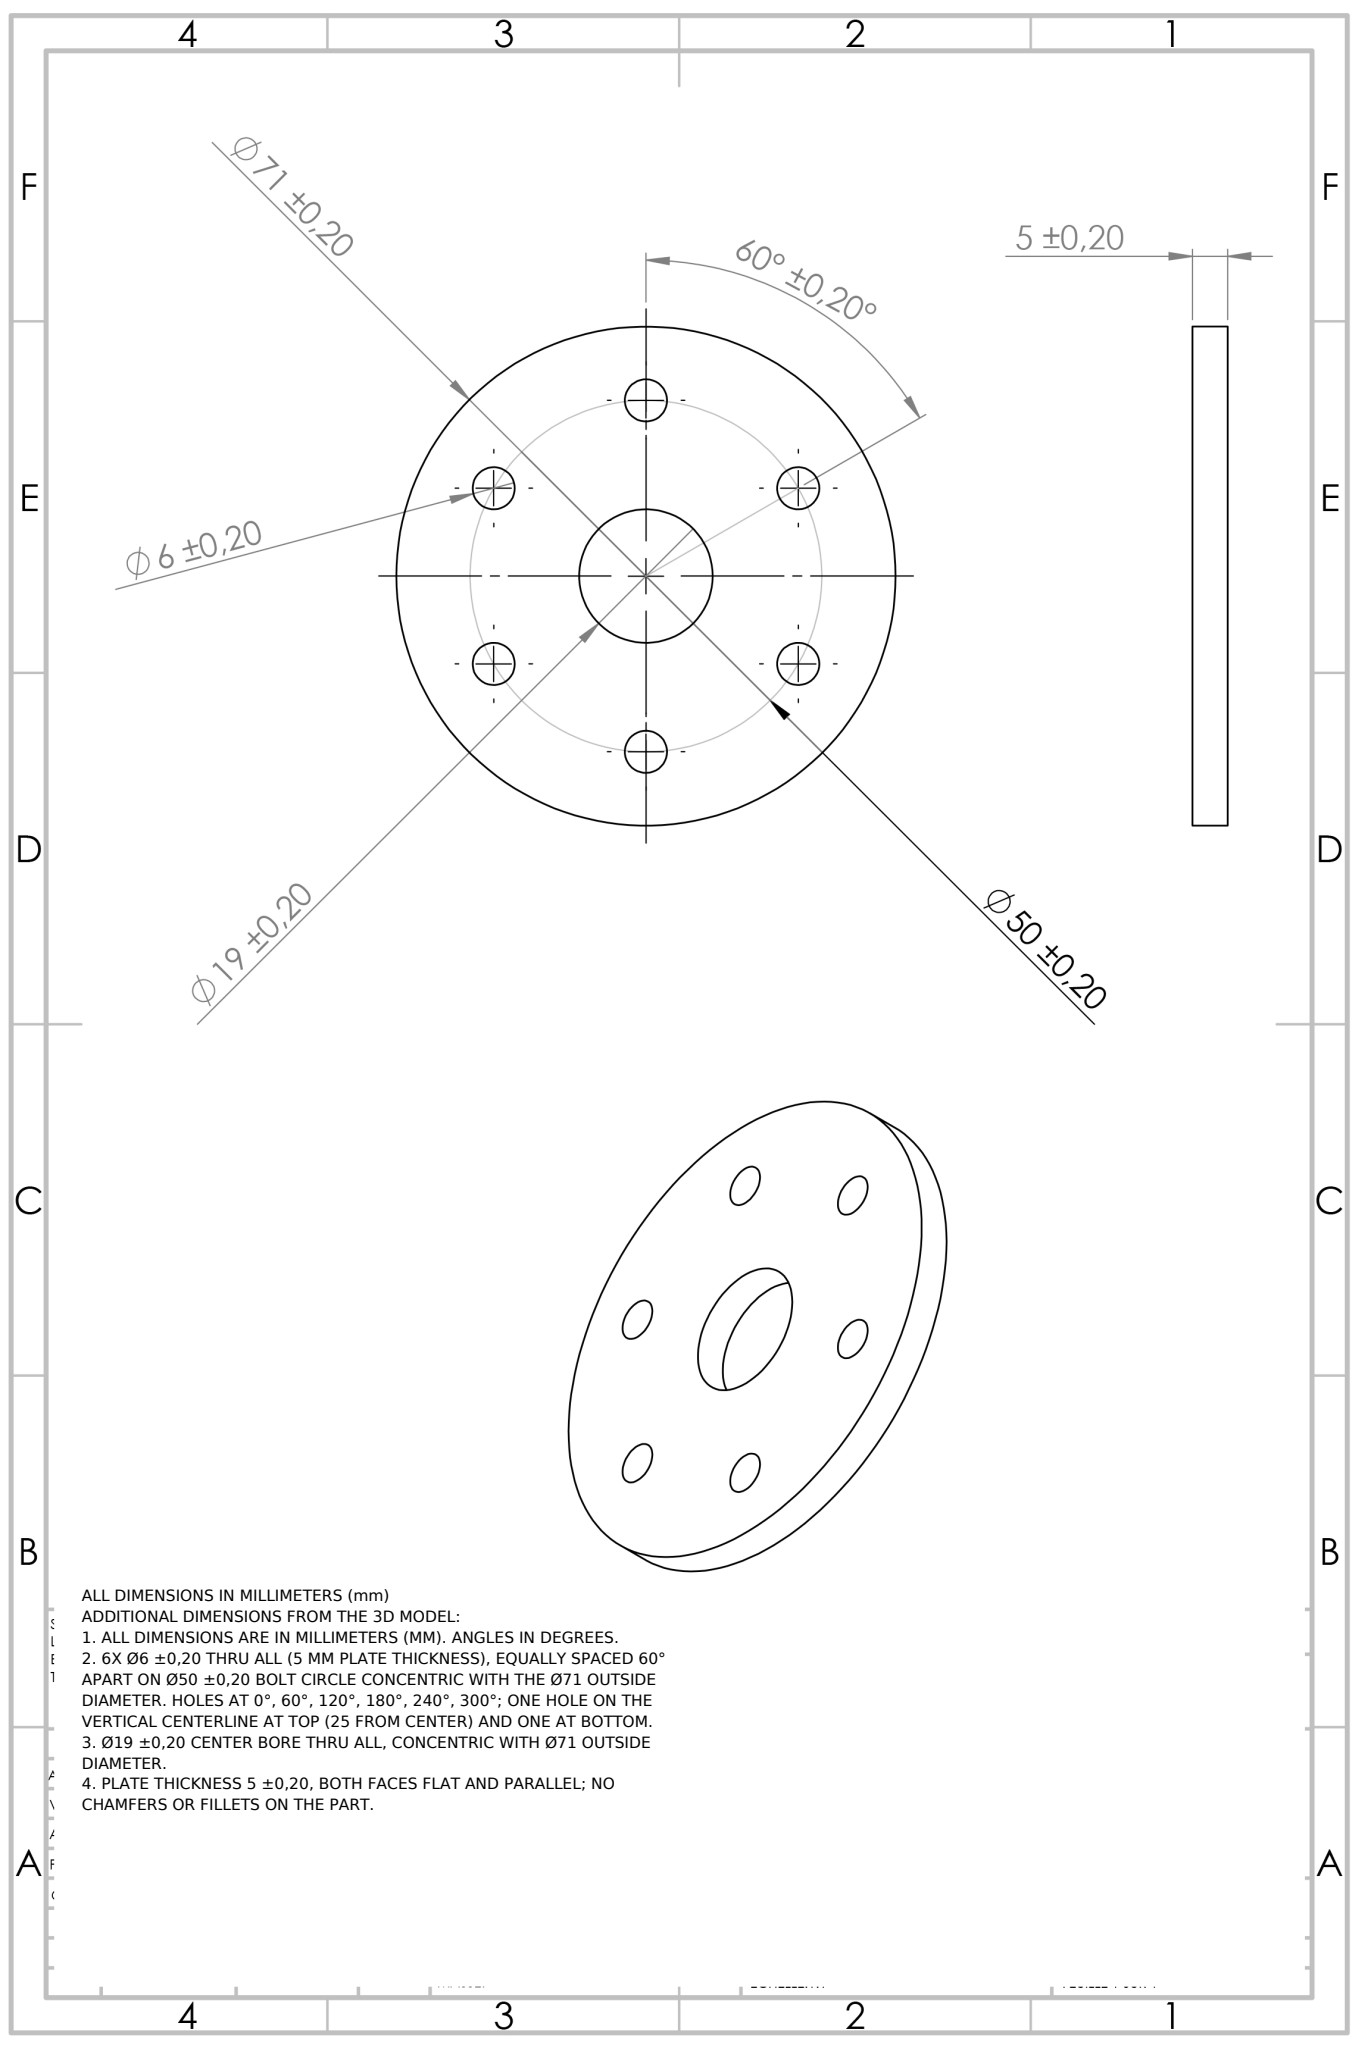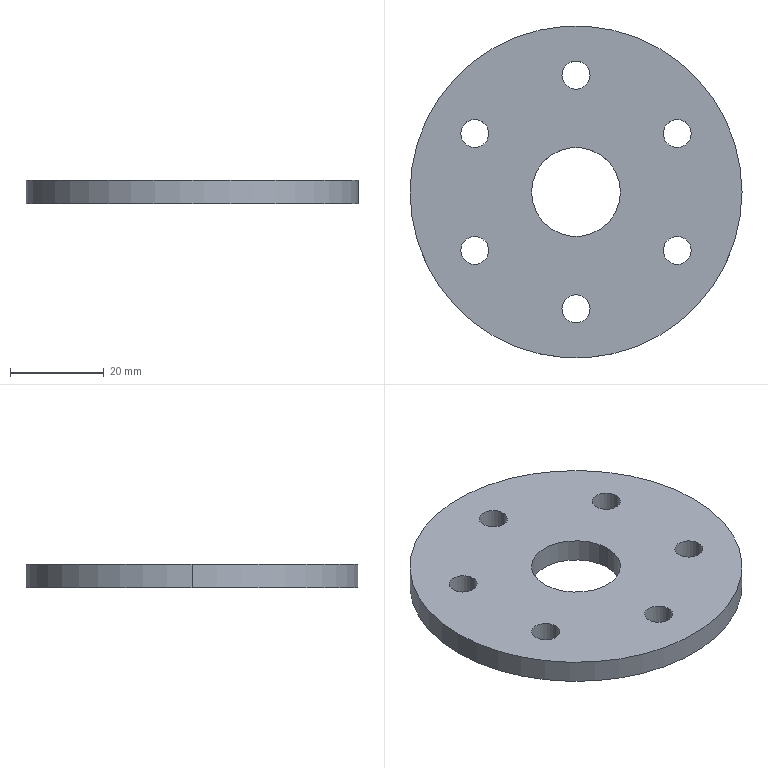Part | NX | mm | 1 solid | 18 faces | box 71 x 71 x 5 mm | volume 17530 mm3 | cylinder 16 | plane 2 | commonest cylinder face diameters 6 x12 19 x2 71 x2
STEP:
#1=COLOUR_RGB('',0.7922,0.8196,0.9333);
#2=FILL_AREA_STYLE_COLOUR('',#1);
#3=FILL_AREA_STYLE('',(#2));
#4=SURFACE_STYLE_FILL_AREA(#3);
#5=SURFACE_SIDE_STYLE('',(#4));
#6=SURFACE_STYLE_USAGE(.BOTH.,#5);
#7=PRESENTATION_STYLE_ASSIGNMENT((#6));
#8=CARTESIAN_POINT('',(-24.651,12.5,5.));
#9=VERTEX_POINT('',#8);
#10=CARTESIAN_POINT('',(-18.651,12.5,5.));
#11=VERTEX_POINT('',#10);
#12=CARTESIAN_POINT('',(-21.651,12.5,5.));
#13=DIRECTION('',(0.,0.,1.));
#14=DIRECTION('',(1.,0.,0.));
#15=AXIS2_PLACEMENT_3D('',#12,#13,#14);
#16=CIRCLE('',#15,3.);
#17=EDGE_CURVE('',#9,#11,#16,.T.);
#18=ORIENTED_EDGE('',*,*,#17,.T.);
#19=CARTESIAN_POINT('',(-18.651,12.5,0.));
#20=VERTEX_POINT('',#19);
#21=CARTESIAN_POINT('',(-18.651,12.5,5.));
#22=DIRECTION('',(0.,0.,-1.));
#23=VECTOR('',#22,1000.);
#24=LINE('',#21,#23);
#25=EDGE_CURVE('',#11,#20,#24,.T.);
#26=ORIENTED_EDGE('',*,*,#25,.T.);
#27=CARTESIAN_POINT('',(-24.651,12.5,0.));
#28=VERTEX_POINT('',#27);
#29=CARTESIAN_POINT('',(-21.651,12.5,0.));
#30=DIRECTION('',(0.,0.,1.));
#31=DIRECTION('',(1.,0.,0.));
#32=AXIS2_PLACEMENT_3D('',#29,#30,#31);
#33=CIRCLE('',#32,3.);
#34=EDGE_CURVE('',#28,#20,#33,.T.);
#35=ORIENTED_EDGE('',*,*,#34,.F.);
#36=CARTESIAN_POINT('',(-24.651,12.5,5.));
#37=DIRECTION('',(0.,0.,-1.));
#38=VECTOR('',#37,1000.);
#39=LINE('',#36,#38);
#40=EDGE_CURVE('',#9,#28,#39,.T.);
#41=ORIENTED_EDGE('',*,*,#40,.F.);
#42=EDGE_LOOP('',(#18,#26,#35,#41));
#43=FACE_OUTER_BOUND('',#42,.T.);
#44=CARTESIAN_POINT('',(-21.651,12.5,5.));
#45=DIRECTION('',(0.,0.,-1.));
#46=DIRECTION('',(-1.,0.,0.));
#47=AXIS2_PLACEMENT_3D('',#44,#45,#46);
#48=CYLINDRICAL_SURFACE('',#47,3.);
#49=ADVANCED_FACE('',(#43),#48,.F.);
#50=CARTESIAN_POINT('',(-24.651,-12.5,5.));
#51=VERTEX_POINT('',#50);
#52=CARTESIAN_POINT('',(-18.651,-12.5,5.));
#53=VERTEX_POINT('',#52);
#54=CARTESIAN_POINT('',(-21.651,-12.5,5.));
#55=DIRECTION('',(0.,0.,1.));
#56=DIRECTION('',(1.,0.,0.));
#57=AXIS2_PLACEMENT_3D('',#54,#55,#56);
#58=CIRCLE('',#57,3.);
#59=EDGE_CURVE('',#51,#53,#58,.T.);
#60=ORIENTED_EDGE('',*,*,#59,.T.);
#61=CARTESIAN_POINT('',(-18.651,-12.5,0.));
#62=VERTEX_POINT('',#61);
#63=CARTESIAN_POINT('',(-18.651,-12.5,5.));
#64=DIRECTION('',(0.,0.,-1.));
#65=VECTOR('',#64,1000.);
#66=LINE('',#63,#65);
#67=EDGE_CURVE('',#53,#62,#66,.T.);
#68=ORIENTED_EDGE('',*,*,#67,.T.);
#69=CARTESIAN_POINT('',(-24.651,-12.5,0.));
#70=VERTEX_POINT('',#69);
#71=CARTESIAN_POINT('',(-21.651,-12.5,0.));
#72=DIRECTION('',(0.,0.,1.));
#73=DIRECTION('',(1.,0.,0.));
#74=AXIS2_PLACEMENT_3D('',#71,#72,#73);
#75=CIRCLE('',#74,3.);
#76=EDGE_CURVE('',#70,#62,#75,.T.);
#77=ORIENTED_EDGE('',*,*,#76,.F.);
#78=CARTESIAN_POINT('',(-24.651,-12.5,5.));
#79=DIRECTION('',(0.,0.,-1.));
#80=VECTOR('',#79,1000.);
#81=LINE('',#78,#80);
#82=EDGE_CURVE('',#51,#70,#81,.T.);
#83=ORIENTED_EDGE('',*,*,#82,.F.);
#84=EDGE_LOOP('',(#60,#68,#77,#83));
#85=FACE_OUTER_BOUND('',#84,.T.);
#86=CARTESIAN_POINT('',(-21.651,-12.5,5.));
#87=DIRECTION('',(0.,0.,-1.));
#88=DIRECTION('',(-1.,0.,0.));
#89=AXIS2_PLACEMENT_3D('',#86,#87,#88);
#90=CYLINDRICAL_SURFACE('',#89,3.);
#91=ADVANCED_FACE('',(#85),#90,.F.);
#92=CARTESIAN_POINT('',(-3.,-25.,5.));
#93=VERTEX_POINT('',#92);
#94=CARTESIAN_POINT('',(3.,-25.,5.));
#95=VERTEX_POINT('',#94);
#96=CARTESIAN_POINT('',(0.,-25.,5.));
#97=DIRECTION('',(0.,0.,1.));
#98=DIRECTION('',(1.,0.,0.));
#99=AXIS2_PLACEMENT_3D('',#96,#97,#98);
#100=CIRCLE('',#99,3.);
#101=EDGE_CURVE('',#93,#95,#100,.T.);
#102=ORIENTED_EDGE('',*,*,#101,.T.);
#103=CARTESIAN_POINT('',(3.,-25.,0.));
#104=VERTEX_POINT('',#103);
#105=CARTESIAN_POINT('',(3.,-25.,5.));
#106=DIRECTION('',(0.,0.,-1.));
#107=VECTOR('',#106,1000.);
#108=LINE('',#105,#107);
#109=EDGE_CURVE('',#95,#104,#108,.T.);
#110=ORIENTED_EDGE('',*,*,#109,.T.);
#111=CARTESIAN_POINT('',(-3.,-25.,0.));
#112=VERTEX_POINT('',#111);
#113=CARTESIAN_POINT('',(0.,-25.,0.));
#114=DIRECTION('',(0.,0.,1.));
#115=DIRECTION('',(1.,0.,0.));
#116=AXIS2_PLACEMENT_3D('',#113,#114,#115);
#117=CIRCLE('',#116,3.);
#118=EDGE_CURVE('',#112,#104,#117,.T.);
#119=ORIENTED_EDGE('',*,*,#118,.F.);
#120=CARTESIAN_POINT('',(-3.,-25.,5.));
#121=DIRECTION('',(0.,0.,-1.));
#122=VECTOR('',#121,1000.);
#123=LINE('',#120,#122);
#124=EDGE_CURVE('',#93,#112,#123,.T.);
#125=ORIENTED_EDGE('',*,*,#124,.F.);
#126=EDGE_LOOP('',(#102,#110,#119,#125));
#127=FACE_OUTER_BOUND('',#126,.T.);
#128=CARTESIAN_POINT('',(0.,-25.,5.));
#129=DIRECTION('',(0.,0.,-1.));
#130=DIRECTION('',(-1.,0.,0.));
#131=AXIS2_PLACEMENT_3D('',#128,#129,#130);
#132=CYLINDRICAL_SURFACE('',#131,3.);
#133=ADVANCED_FACE('',(#127),#132,.F.);
#134=CARTESIAN_POINT('',(18.651,-12.5,5.));
#135=VERTEX_POINT('',#134);
#136=CARTESIAN_POINT('',(24.651,-12.5,5.));
#137=VERTEX_POINT('',#136);
#138=CARTESIAN_POINT('',(21.651,-12.5,5.));
#139=DIRECTION('',(0.,0.,1.));
#140=DIRECTION('',(1.,0.,0.));
#141=AXIS2_PLACEMENT_3D('',#138,#139,#140);
#142=CIRCLE('',#141,3.);
#143=EDGE_CURVE('',#135,#137,#142,.T.);
#144=ORIENTED_EDGE('',*,*,#143,.T.);
#145=CARTESIAN_POINT('',(24.651,-12.5,0.));
#146=VERTEX_POINT('',#145);
#147=CARTESIAN_POINT('',(24.651,-12.5,5.));
#148=DIRECTION('',(0.,0.,-1.));
#149=VECTOR('',#148,1000.);
#150=LINE('',#147,#149);
#151=EDGE_CURVE('',#137,#146,#150,.T.);
#152=ORIENTED_EDGE('',*,*,#151,.T.);
#153=CARTESIAN_POINT('',(18.651,-12.5,0.));
#154=VERTEX_POINT('',#153);
#155=CARTESIAN_POINT('',(21.651,-12.5,0.));
#156=DIRECTION('',(0.,0.,1.));
#157=DIRECTION('',(1.,0.,0.));
#158=AXIS2_PLACEMENT_3D('',#155,#156,#157);
#159=CIRCLE('',#158,3.);
#160=EDGE_CURVE('',#154,#146,#159,.T.);
#161=ORIENTED_EDGE('',*,*,#160,.F.);
#162=CARTESIAN_POINT('',(18.651,-12.5,5.));
#163=DIRECTION('',(0.,0.,-1.));
#164=VECTOR('',#163,1000.);
#165=LINE('',#162,#164);
#166=EDGE_CURVE('',#135,#154,#165,.T.);
#167=ORIENTED_EDGE('',*,*,#166,.F.);
#168=EDGE_LOOP('',(#144,#152,#161,#167));
#169=FACE_OUTER_BOUND('',#168,.T.);
#170=CARTESIAN_POINT('',(21.651,-12.5,5.));
#171=DIRECTION('',(0.,0.,-1.));
#172=DIRECTION('',(-1.,0.,0.));
#173=AXIS2_PLACEMENT_3D('',#170,#171,#172);
#174=CYLINDRICAL_SURFACE('',#173,3.);
#175=ADVANCED_FACE('',(#169),#174,.F.);
#176=CARTESIAN_POINT('',(18.651,12.5,5.));
#177=VERTEX_POINT('',#176);
#178=CARTESIAN_POINT('',(24.651,12.5,5.));
#179=VERTEX_POINT('',#178);
#180=CARTESIAN_POINT('',(21.651,12.5,5.));
#181=DIRECTION('',(0.,0.,1.));
#182=DIRECTION('',(1.,0.,0.));
#183=AXIS2_PLACEMENT_3D('',#180,#181,#182);
#184=CIRCLE('',#183,3.);
#185=EDGE_CURVE('',#177,#179,#184,.T.);
#186=ORIENTED_EDGE('',*,*,#185,.T.);
#187=CARTESIAN_POINT('',(24.651,12.5,0.));
#188=VERTEX_POINT('',#187);
#189=CARTESIAN_POINT('',(24.651,12.5,5.));
#190=DIRECTION('',(0.,0.,-1.));
#191=VECTOR('',#190,1000.);
#192=LINE('',#189,#191);
#193=EDGE_CURVE('',#179,#188,#192,.T.);
#194=ORIENTED_EDGE('',*,*,#193,.T.);
#195=CARTESIAN_POINT('',(18.651,12.5,0.));
#196=VERTEX_POINT('',#195);
#197=CARTESIAN_POINT('',(21.651,12.5,0.));
#198=DIRECTION('',(0.,0.,1.));
#199=DIRECTION('',(1.,0.,0.));
#200=AXIS2_PLACEMENT_3D('',#197,#198,#199);
#201=CIRCLE('',#200,3.);
#202=EDGE_CURVE('',#196,#188,#201,.T.);
#203=ORIENTED_EDGE('',*,*,#202,.F.);
#204=CARTESIAN_POINT('',(18.651,12.5,5.));
#205=DIRECTION('',(0.,0.,-1.));
#206=VECTOR('',#205,1000.);
#207=LINE('',#204,#206);
#208=EDGE_CURVE('',#177,#196,#207,.T.);
#209=ORIENTED_EDGE('',*,*,#208,.F.);
#210=EDGE_LOOP('',(#186,#194,#203,#209));
#211=FACE_OUTER_BOUND('',#210,.T.);
#212=CARTESIAN_POINT('',(21.651,12.5,5.));
#213=DIRECTION('',(0.,0.,-1.));
#214=DIRECTION('',(-1.,0.,0.));
#215=AXIS2_PLACEMENT_3D('',#212,#213,#214);
#216=CYLINDRICAL_SURFACE('',#215,3.);
#217=ADVANCED_FACE('',(#211),#216,.F.);
#218=CARTESIAN_POINT('',(-3.,25.,5.));
#219=VERTEX_POINT('',#218);
#220=CARTESIAN_POINT('',(3.,25.,5.));
#221=VERTEX_POINT('',#220);
#222=CARTESIAN_POINT('',(0.,25.,5.));
#223=DIRECTION('',(0.,0.,1.));
#224=DIRECTION('',(1.,0.,0.));
#225=AXIS2_PLACEMENT_3D('',#222,#223,#224);
#226=CIRCLE('',#225,3.);
#227=EDGE_CURVE('',#219,#221,#226,.T.);
#228=ORIENTED_EDGE('',*,*,#227,.T.);
#229=CARTESIAN_POINT('',(3.,25.,0.));
#230=VERTEX_POINT('',#229);
#231=CARTESIAN_POINT('',(3.,25.,5.));
#232=DIRECTION('',(0.,0.,-1.));
#233=VECTOR('',#232,1000.);
#234=LINE('',#231,#233);
#235=EDGE_CURVE('',#221,#230,#234,.T.);
#236=ORIENTED_EDGE('',*,*,#235,.T.);
#237=CARTESIAN_POINT('',(-3.,25.,0.));
#238=VERTEX_POINT('',#237);
#239=CARTESIAN_POINT('',(0.,25.,0.));
#240=DIRECTION('',(0.,0.,1.));
#241=DIRECTION('',(1.,0.,0.));
#242=AXIS2_PLACEMENT_3D('',#239,#240,#241);
#243=CIRCLE('',#242,3.);
#244=EDGE_CURVE('',#238,#230,#243,.T.);
#245=ORIENTED_EDGE('',*,*,#244,.F.);
#246=CARTESIAN_POINT('',(-3.,25.,5.));
#247=DIRECTION('',(0.,0.,-1.));
#248=VECTOR('',#247,1000.);
#249=LINE('',#246,#248);
#250=EDGE_CURVE('',#219,#238,#249,.T.);
#251=ORIENTED_EDGE('',*,*,#250,.F.);
#252=EDGE_LOOP('',(#228,#236,#245,#251));
#253=FACE_OUTER_BOUND('',#252,.T.);
#254=CARTESIAN_POINT('',(0.,25.,5.));
#255=DIRECTION('',(0.,0.,-1.));
#256=DIRECTION('',(-1.,0.,0.));
#257=AXIS2_PLACEMENT_3D('',#254,#255,#256);
#258=CYLINDRICAL_SURFACE('',#257,3.);
#259=ADVANCED_FACE('',(#253),#258,.F.);
#260=CARTESIAN_POINT('',(-9.5,0.,5.));
#261=VERTEX_POINT('',#260);
#262=CARTESIAN_POINT('',(9.5,0.,5.));
#263=VERTEX_POINT('',#262);
#264=CARTESIAN_POINT('',(0.,0.,5.));
#265=DIRECTION('',(0.,0.,1.));
#266=DIRECTION('',(1.,0.,0.));
#267=AXIS2_PLACEMENT_3D('',#264,#265,#266);
#268=CIRCLE('',#267,9.5);
#269=EDGE_CURVE('',#261,#263,#268,.T.);
#270=ORIENTED_EDGE('',*,*,#269,.T.);
#271=CARTESIAN_POINT('',(9.5,0.,0.));
#272=VERTEX_POINT('',#271);
#273=CARTESIAN_POINT('',(9.5,0.,5.));
#274=DIRECTION('',(0.,0.,-1.));
#275=VECTOR('',#274,1000.);
#276=LINE('',#273,#275);
#277=EDGE_CURVE('',#263,#272,#276,.T.);
#278=ORIENTED_EDGE('',*,*,#277,.T.);
#279=CARTESIAN_POINT('',(-9.5,0.,0.));
#280=VERTEX_POINT('',#279);
#281=CARTESIAN_POINT('',(0.,0.,0.));
#282=DIRECTION('',(0.,0.,1.));
#283=DIRECTION('',(1.,0.,0.));
#284=AXIS2_PLACEMENT_3D('',#281,#282,#283);
#285=CIRCLE('',#284,9.5);
#286=EDGE_CURVE('',#280,#272,#285,.T.);
#287=ORIENTED_EDGE('',*,*,#286,.F.);
#288=CARTESIAN_POINT('',(-9.5,0.,5.));
#289=DIRECTION('',(0.,0.,-1.));
#290=VECTOR('',#289,1000.);
#291=LINE('',#288,#290);
#292=EDGE_CURVE('',#261,#280,#291,.T.);
#293=ORIENTED_EDGE('',*,*,#292,.F.);
#294=EDGE_LOOP('',(#270,#278,#287,#293));
#295=FACE_OUTER_BOUND('',#294,.T.);
#296=CARTESIAN_POINT('',(0.,0.,5.));
#297=DIRECTION('',(0.,0.,-1.));
#298=DIRECTION('',(-1.,0.,0.));
#299=AXIS2_PLACEMENT_3D('',#296,#297,#298);
#300=CYLINDRICAL_SURFACE('',#299,9.5);
#301=ADVANCED_FACE('',(#295),#300,.F.);
#302=CARTESIAN_POINT('',(35.5,0.,5.));
#303=VERTEX_POINT('',#302);
#304=CARTESIAN_POINT('',(-35.5,0.,5.));
#305=VERTEX_POINT('',#304);
#306=CARTESIAN_POINT('',(0.,0.,5.));
#307=DIRECTION('',(0.,0.,1.));
#308=DIRECTION('',(1.,0.,0.));
#309=AXIS2_PLACEMENT_3D('',#306,#307,#308);
#310=CIRCLE('',#309,35.5);
#311=EDGE_CURVE('',#303,#305,#310,.T.);
#312=ORIENTED_EDGE('',*,*,#311,.F.);
#313=CARTESIAN_POINT('',(35.5,0.,0.));
#314=VERTEX_POINT('',#313);
#315=CARTESIAN_POINT('',(35.5,0.,5.));
#316=DIRECTION('',(0.,0.,-1.));
#317=VECTOR('',#316,1000.);
#318=LINE('',#315,#317);
#319=EDGE_CURVE('',#303,#314,#318,.T.);
#320=ORIENTED_EDGE('',*,*,#319,.T.);
#321=CARTESIAN_POINT('',(-35.5,0.,0.));
#322=VERTEX_POINT('',#321);
#323=CARTESIAN_POINT('',(0.,0.,0.));
#324=DIRECTION('',(0.,0.,1.));
#325=DIRECTION('',(1.,0.,0.));
#326=AXIS2_PLACEMENT_3D('',#323,#324,#325);
#327=CIRCLE('',#326,35.5);
#328=EDGE_CURVE('',#314,#322,#327,.T.);
#329=ORIENTED_EDGE('',*,*,#328,.T.);
#330=CARTESIAN_POINT('',(-35.5,0.,5.));
#331=DIRECTION('',(0.,0.,-1.));
#332=VECTOR('',#331,1000.);
#333=LINE('',#330,#332);
#334=EDGE_CURVE('',#305,#322,#333,.T.);
#335=ORIENTED_EDGE('',*,*,#334,.F.);
#336=EDGE_LOOP('',(#312,#320,#329,#335));
#337=FACE_OUTER_BOUND('',#336,.T.);
#338=CARTESIAN_POINT('',(0.,0.,5.));
#339=DIRECTION('',(0.,0.,-1.));
#340=DIRECTION('',(-1.,0.,0.));
#341=AXIS2_PLACEMENT_3D('',#338,#339,#340);
#342=CYLINDRICAL_SURFACE('',#341,35.5);
#343=ADVANCED_FACE('',(#337),#342,.T.);
#344=ORIENTED_EDGE('',*,*,#59,.F.);
#345=CARTESIAN_POINT('',(-21.651,-12.5,5.));
#346=DIRECTION('',(0.,0.,1.));
#347=DIRECTION('',(1.,0.,0.));
#348=AXIS2_PLACEMENT_3D('',#345,#346,#347);
#349=CIRCLE('',#348,3.);
#350=EDGE_CURVE('',#53,#51,#349,.T.);
#351=ORIENTED_EDGE('',*,*,#350,.F.);
#352=EDGE_LOOP('',(#344,#351));
#353=FACE_BOUND('',#352,.T.);
#354=ORIENTED_EDGE('',*,*,#143,.F.);
#355=CARTESIAN_POINT('',(21.651,-12.5,5.));
#356=DIRECTION('',(0.,0.,1.));
#357=DIRECTION('',(1.,0.,0.));
#358=AXIS2_PLACEMENT_3D('',#355,#356,#357);
#359=CIRCLE('',#358,3.);
#360=EDGE_CURVE('',#137,#135,#359,.T.);
#361=ORIENTED_EDGE('',*,*,#360,.F.);
#362=EDGE_LOOP('',(#354,#361));
#363=FACE_BOUND('',#362,.T.);
#364=ORIENTED_EDGE('',*,*,#227,.F.);
#365=CARTESIAN_POINT('',(0.,25.,5.));
#366=DIRECTION('',(0.,0.,1.));
#367=DIRECTION('',(1.,0.,0.));
#368=AXIS2_PLACEMENT_3D('',#365,#366,#367);
#369=CIRCLE('',#368,3.);
#370=EDGE_CURVE('',#221,#219,#369,.T.);
#371=ORIENTED_EDGE('',*,*,#370,.F.);
#372=EDGE_LOOP('',(#364,#371));
#373=FACE_BOUND('',#372,.T.);
#374=CARTESIAN_POINT('',(0.,0.,5.));
#375=DIRECTION('',(0.,0.,1.));
#376=DIRECTION('',(1.,0.,0.));
#377=AXIS2_PLACEMENT_3D('',#374,#375,#376);
#378=CIRCLE('',#377,35.5);
#379=EDGE_CURVE('',#305,#303,#378,.T.);
#380=ORIENTED_EDGE('',*,*,#379,.T.);
#381=ORIENTED_EDGE('',*,*,#311,.T.);
#382=EDGE_LOOP('',(#380,#381));
#383=FACE_OUTER_BOUND('',#382,.T.);
#384=ORIENTED_EDGE('',*,*,#269,.F.);
#385=CARTESIAN_POINT('',(0.,0.,5.));
#386=DIRECTION('',(0.,0.,1.));
#387=DIRECTION('',(1.,0.,0.));
#388=AXIS2_PLACEMENT_3D('',#385,#386,#387);
#389=CIRCLE('',#388,9.5);
#390=EDGE_CURVE('',#263,#261,#389,.T.);
#391=ORIENTED_EDGE('',*,*,#390,.F.);
#392=EDGE_LOOP('',(#384,#391));
#393=FACE_BOUND('',#392,.T.);
#394=ORIENTED_EDGE('',*,*,#185,.F.);
#395=CARTESIAN_POINT('',(21.651,12.5,5.));
#396=DIRECTION('',(0.,0.,1.));
#397=DIRECTION('',(1.,0.,0.));
#398=AXIS2_PLACEMENT_3D('',#395,#396,#397);
#399=CIRCLE('',#398,3.);
#400=EDGE_CURVE('',#179,#177,#399,.T.);
#401=ORIENTED_EDGE('',*,*,#400,.F.);
#402=EDGE_LOOP('',(#394,#401));
#403=FACE_BOUND('',#402,.T.);
#404=ORIENTED_EDGE('',*,*,#101,.F.);
#405=CARTESIAN_POINT('',(0.,-25.,5.));
#406=DIRECTION('',(0.,0.,1.));
#407=DIRECTION('',(1.,0.,0.));
#408=AXIS2_PLACEMENT_3D('',#405,#406,#407);
#409=CIRCLE('',#408,3.);
#410=EDGE_CURVE('',#95,#93,#409,.T.);
#411=ORIENTED_EDGE('',*,*,#410,.F.);
#412=EDGE_LOOP('',(#404,#411));
#413=FACE_BOUND('',#412,.T.);
#414=ORIENTED_EDGE('',*,*,#17,.F.);
#415=CARTESIAN_POINT('',(-21.651,12.5,5.));
#416=DIRECTION('',(0.,0.,1.));
#417=DIRECTION('',(1.,0.,0.));
#418=AXIS2_PLACEMENT_3D('',#415,#416,#417);
#419=CIRCLE('',#418,3.);
#420=EDGE_CURVE('',#11,#9,#419,.T.);
#421=ORIENTED_EDGE('',*,*,#420,.F.);
#422=EDGE_LOOP('',(#414,#421));
#423=FACE_BOUND('',#422,.T.);
#424=CARTESIAN_POINT('',(0.,0.,5.));
#425=DIRECTION('',(0.,0.,1.));
#426=DIRECTION('',(1.,0.,0.));
#427=AXIS2_PLACEMENT_3D('',#424,#425,#426);
#428=PLANE('',#427);
#429=ADVANCED_FACE('',(#353,#363,#373,#383,#393,#403,#413,#423),#428,.T.);
#430=CARTESIAN_POINT('',(0.,0.,0.));
#431=DIRECTION('',(0.,0.,1.));
#432=DIRECTION('',(1.,0.,0.));
#433=AXIS2_PLACEMENT_3D('',#430,#431,#432);
#434=CIRCLE('',#433,35.5);
#435=EDGE_CURVE('',#322,#314,#434,.T.);
#436=ORIENTED_EDGE('',*,*,#435,.F.);
#437=ORIENTED_EDGE('',*,*,#328,.F.);
#438=EDGE_LOOP('',(#436,#437));
#439=FACE_OUTER_BOUND('',#438,.T.);
#440=ORIENTED_EDGE('',*,*,#286,.T.);
#441=CARTESIAN_POINT('',(0.,0.,0.));
#442=DIRECTION('',(0.,0.,1.));
#443=DIRECTION('',(1.,0.,0.));
#444=AXIS2_PLACEMENT_3D('',#441,#442,#443);
#445=CIRCLE('',#444,9.5);
#446=EDGE_CURVE('',#272,#280,#445,.T.);
#447=ORIENTED_EDGE('',*,*,#446,.T.);
#448=EDGE_LOOP('',(#440,#447));
#449=FACE_BOUND('',#448,.T.);
#450=ORIENTED_EDGE('',*,*,#244,.T.);
#451=CARTESIAN_POINT('',(0.,25.,0.));
#452=DIRECTION('',(0.,0.,1.));
#453=DIRECTION('',(1.,0.,0.));
#454=AXIS2_PLACEMENT_3D('',#451,#452,#453);
#455=CIRCLE('',#454,3.);
#456=EDGE_CURVE('',#230,#238,#455,.T.);
#457=ORIENTED_EDGE('',*,*,#456,.T.);
#458=EDGE_LOOP('',(#450,#457));
#459=FACE_BOUND('',#458,.T.);
#460=ORIENTED_EDGE('',*,*,#202,.T.);
#461=CARTESIAN_POINT('',(21.651,12.5,0.));
#462=DIRECTION('',(0.,0.,1.));
#463=DIRECTION('',(1.,0.,0.));
#464=AXIS2_PLACEMENT_3D('',#461,#462,#463);
#465=CIRCLE('',#464,3.);
#466=EDGE_CURVE('',#188,#196,#465,.T.);
#467=ORIENTED_EDGE('',*,*,#466,.T.);
#468=EDGE_LOOP('',(#460,#467));
#469=FACE_BOUND('',#468,.T.);
#470=ORIENTED_EDGE('',*,*,#160,.T.);
#471=CARTESIAN_POINT('',(21.651,-12.5,0.));
#472=DIRECTION('',(0.,0.,1.));
#473=DIRECTION('',(1.,0.,0.));
#474=AXIS2_PLACEMENT_3D('',#471,#472,#473);
#475=CIRCLE('',#474,3.);
#476=EDGE_CURVE('',#146,#154,#475,.T.);
#477=ORIENTED_EDGE('',*,*,#476,.T.);
#478=EDGE_LOOP('',(#470,#477));
#479=FACE_BOUND('',#478,.T.);
#480=ORIENTED_EDGE('',*,*,#118,.T.);
#481=CARTESIAN_POINT('',(0.,-25.,0.));
#482=DIRECTION('',(0.,0.,1.));
#483=DIRECTION('',(1.,0.,0.));
#484=AXIS2_PLACEMENT_3D('',#481,#482,#483);
#485=CIRCLE('',#484,3.);
#486=EDGE_CURVE('',#104,#112,#485,.T.);
#487=ORIENTED_EDGE('',*,*,#486,.T.);
#488=EDGE_LOOP('',(#480,#487));
#489=FACE_BOUND('',#488,.T.);
#490=ORIENTED_EDGE('',*,*,#76,.T.);
#491=CARTESIAN_POINT('',(-21.651,-12.5,0.));
#492=DIRECTION('',(0.,0.,1.));
#493=DIRECTION('',(1.,0.,0.));
#494=AXIS2_PLACEMENT_3D('',#491,#492,#493);
#495=CIRCLE('',#494,3.);
#496=EDGE_CURVE('',#62,#70,#495,.T.);
#497=ORIENTED_EDGE('',*,*,#496,.T.);
#498=EDGE_LOOP('',(#490,#497));
#499=FACE_BOUND('',#498,.T.);
#500=ORIENTED_EDGE('',*,*,#34,.T.);
#501=CARTESIAN_POINT('',(-21.651,12.5,0.));
#502=DIRECTION('',(0.,0.,1.));
#503=DIRECTION('',(1.,0.,0.));
#504=AXIS2_PLACEMENT_3D('',#501,#502,#503);
#505=CIRCLE('',#504,3.);
#506=EDGE_CURVE('',#20,#28,#505,.T.);
#507=ORIENTED_EDGE('',*,*,#506,.T.);
#508=EDGE_LOOP('',(#500,#507));
#509=FACE_BOUND('',#508,.T.);
#510=CARTESIAN_POINT('',(0.,0.,0.));
#511=DIRECTION('',(0.,0.,1.));
#512=DIRECTION('',(1.,0.,0.));
#513=AXIS2_PLACEMENT_3D('',#510,#511,#512);
#514=PLANE('',#513);
#515=ADVANCED_FACE('',(#439,#449,#459,#469,#479,#489,#499,#509),#514,.F.);
#516=ORIENTED_EDGE('',*,*,#319,.F.);
#517=ORIENTED_EDGE('',*,*,#379,.F.);
#518=ORIENTED_EDGE('',*,*,#334,.T.);
#519=ORIENTED_EDGE('',*,*,#435,.T.);
#520=EDGE_LOOP('',(#516,#517,#518,#519));
#521=FACE_OUTER_BOUND('',#520,.T.);
#522=CARTESIAN_POINT('',(0.,0.,5.));
#523=DIRECTION('',(0.,0.,-1.));
#524=DIRECTION('',(-1.,0.,0.));
#525=AXIS2_PLACEMENT_3D('',#522,#523,#524);
#526=CYLINDRICAL_SURFACE('',#525,35.5);
#527=ADVANCED_FACE('',(#521),#526,.T.);
#528=ORIENTED_EDGE('',*,*,#277,.F.);
#529=ORIENTED_EDGE('',*,*,#390,.T.);
#530=ORIENTED_EDGE('',*,*,#292,.T.);
#531=ORIENTED_EDGE('',*,*,#446,.F.);
#532=EDGE_LOOP('',(#528,#529,#530,#531));
#533=FACE_OUTER_BOUND('',#532,.T.);
#534=CARTESIAN_POINT('',(0.,0.,5.));
#535=DIRECTION('',(0.,0.,-1.));
#536=DIRECTION('',(-1.,0.,0.));
#537=AXIS2_PLACEMENT_3D('',#534,#535,#536);
#538=CYLINDRICAL_SURFACE('',#537,9.5);
#539=ADVANCED_FACE('',(#533),#538,.F.);
#540=ORIENTED_EDGE('',*,*,#235,.F.);
#541=ORIENTED_EDGE('',*,*,#370,.T.);
#542=ORIENTED_EDGE('',*,*,#250,.T.);
#543=ORIENTED_EDGE('',*,*,#456,.F.);
#544=EDGE_LOOP('',(#540,#541,#542,#543));
#545=FACE_OUTER_BOUND('',#544,.T.);
#546=CARTESIAN_POINT('',(0.,25.,5.));
#547=DIRECTION('',(0.,0.,-1.));
#548=DIRECTION('',(-1.,0.,0.));
#549=AXIS2_PLACEMENT_3D('',#546,#547,#548);
#550=CYLINDRICAL_SURFACE('',#549,3.);
#551=ADVANCED_FACE('',(#545),#550,.F.);
#552=ORIENTED_EDGE('',*,*,#193,.F.);
#553=ORIENTED_EDGE('',*,*,#400,.T.);
#554=ORIENTED_EDGE('',*,*,#208,.T.);
#555=ORIENTED_EDGE('',*,*,#466,.F.);
#556=EDGE_LOOP('',(#552,#553,#554,#555));
#557=FACE_OUTER_BOUND('',#556,.T.);
#558=CARTESIAN_POINT('',(21.651,12.5,5.));
#559=DIRECTION('',(0.,0.,-1.));
#560=DIRECTION('',(-1.,0.,0.));
#561=AXIS2_PLACEMENT_3D('',#558,#559,#560);
#562=CYLINDRICAL_SURFACE('',#561,3.);
#563=ADVANCED_FACE('',(#557),#562,.F.);
#564=ORIENTED_EDGE('',*,*,#151,.F.);
#565=ORIENTED_EDGE('',*,*,#360,.T.);
#566=ORIENTED_EDGE('',*,*,#166,.T.);
#567=ORIENTED_EDGE('',*,*,#476,.F.);
#568=EDGE_LOOP('',(#564,#565,#566,#567));
#569=FACE_OUTER_BOUND('',#568,.T.);
#570=CARTESIAN_POINT('',(21.651,-12.5,5.));
#571=DIRECTION('',(0.,0.,-1.));
#572=DIRECTION('',(-1.,0.,0.));
#573=AXIS2_PLACEMENT_3D('',#570,#571,#572);
#574=CYLINDRICAL_SURFACE('',#573,3.);
#575=ADVANCED_FACE('',(#569),#574,.F.);
#576=ORIENTED_EDGE('',*,*,#109,.F.);
#577=ORIENTED_EDGE('',*,*,#410,.T.);
#578=ORIENTED_EDGE('',*,*,#124,.T.);
#579=ORIENTED_EDGE('',*,*,#486,.F.);
#580=EDGE_LOOP('',(#576,#577,#578,#579));
#581=FACE_OUTER_BOUND('',#580,.T.);
#582=CARTESIAN_POINT('',(0.,-25.,5.));
#583=DIRECTION('',(0.,0.,-1.));
#584=DIRECTION('',(-1.,0.,0.));
#585=AXIS2_PLACEMENT_3D('',#582,#583,#584);
#586=CYLINDRICAL_SURFACE('',#585,3.);
#587=ADVANCED_FACE('',(#581),#586,.F.);
#588=ORIENTED_EDGE('',*,*,#67,.F.);
#589=ORIENTED_EDGE('',*,*,#350,.T.);
#590=ORIENTED_EDGE('',*,*,#82,.T.);
#591=ORIENTED_EDGE('',*,*,#496,.F.);
#592=EDGE_LOOP('',(#588,#589,#590,#591));
#593=FACE_OUTER_BOUND('',#592,.T.);
#594=CARTESIAN_POINT('',(-21.651,-12.5,5.));
#595=DIRECTION('',(0.,0.,-1.));
#596=DIRECTION('',(-1.,0.,0.));
#597=AXIS2_PLACEMENT_3D('',#594,#595,#596);
#598=CYLINDRICAL_SURFACE('',#597,3.);
#599=ADVANCED_FACE('',(#593),#598,.F.);
#600=ORIENTED_EDGE('',*,*,#25,.F.);
#601=ORIENTED_EDGE('',*,*,#420,.T.);
#602=ORIENTED_EDGE('',*,*,#40,.T.);
#603=ORIENTED_EDGE('',*,*,#506,.F.);
#604=EDGE_LOOP('',(#600,#601,#602,#603));
#605=FACE_OUTER_BOUND('',#604,.T.);
#606=CARTESIAN_POINT('',(-21.651,12.5,5.));
#607=DIRECTION('',(0.,0.,-1.));
#608=DIRECTION('',(-1.,0.,0.));
#609=AXIS2_PLACEMENT_3D('',#606,#607,#608);
#610=CYLINDRICAL_SURFACE('',#609,3.);
#611=ADVANCED_FACE('',(#605),#610,.F.);
#612=CLOSED_SHELL('',(#49,#91,#133,#175,#217,#259,#301,#343,#429,#515,#527,#539,#551,#563,#575,#587,#599,#611));
#613=MANIFOLD_SOLID_BREP('',#612);
#614=CARTESIAN_POINT('',(0.,0.,0.));
#615=DIRECTION('',(0.,0.,1.));
#616=DIRECTION('',(1.,0.,0.));
#617=AXIS2_PLACEMENT_3D('',#614,#615,#616);
#618=(LENGTH_UNIT()NAMED_UNIT(*)SI_UNIT(.MILLI.,.METRE.));
#619=UNCERTAINTY_MEASURE_WITH_UNIT(LENGTH_MEASURE(0.00001),#618,'','');
#620=(NAMED_UNIT(*)PLANE_ANGLE_UNIT()SI_UNIT($,.RADIAN.));
#621=(NAMED_UNIT(*)SI_UNIT($,.STERADIAN.)SOLID_ANGLE_UNIT());
#622=(GEOMETRIC_REPRESENTATION_CONTEXT(3)GLOBAL_UNCERTAINTY_ASSIGNED_CONTEXT((#619))GLOBAL_UNIT_ASSIGNED_CONTEXT((#618,#620,#621))REPRESENTATION_CONTEXT('',''));
#623=ADVANCED_BREP_SHAPE_REPRESENTATION('',(#613,#617),#622);
#624=STYLED_ITEM('',(#7),#623);
#625=PRESENTATION_LAYER_ASSIGNMENT('','',(#624));
#626=(LENGTH_UNIT()NAMED_UNIT(*)SI_UNIT(.MILLI.,.METRE.));
#627=UNCERTAINTY_MEASURE_WITH_UNIT(LENGTH_MEASURE(0.00001),#626,'','');
#628=(NAMED_UNIT(*)PLANE_ANGLE_UNIT()SI_UNIT($,.RADIAN.));
#629=(NAMED_UNIT(*)SI_UNIT($,.STERADIAN.)SOLID_ANGLE_UNIT());
#630=(GEOMETRIC_REPRESENTATION_CONTEXT(3)GLOBAL_UNCERTAINTY_ASSIGNED_CONTEXT((#627))GLOBAL_UNIT_ASSIGNED_CONTEXT((#626,#628,#629))REPRESENTATION_CONTEXT('',''));
#631=MECHANICAL_DESIGN_GEOMETRIC_PRESENTATION_REPRESENTATION('',(#624),#630);
#632=COLOUR_RGB('',0.7922,0.8196,0.9333);
#633=FILL_AREA_STYLE_COLOUR('',#632);
#634=FILL_AREA_STYLE('',(#633));
#635=SURFACE_STYLE_FILL_AREA(#634);
#636=SURFACE_SIDE_STYLE('',(#635));
#637=SURFACE_STYLE_USAGE(.BOTH.,#636);
#638=PRESENTATION_STYLE_ASSIGNMENT((#637));
#639=STYLED_ITEM('',(#638),#613);
#640=PRESENTATION_LAYER_ASSIGNMENT('','',(#639));
#641=(LENGTH_UNIT()NAMED_UNIT(*)SI_UNIT(.MILLI.,.METRE.));
#642=UNCERTAINTY_MEASURE_WITH_UNIT(LENGTH_MEASURE(0.00001),#641,'','');
#643=(NAMED_UNIT(*)PLANE_ANGLE_UNIT()SI_UNIT($,.RADIAN.));
#644=(NAMED_UNIT(*)SI_UNIT($,.STERADIAN.)SOLID_ANGLE_UNIT());
#645=(GEOMETRIC_REPRESENTATION_CONTEXT(3)GLOBAL_UNCERTAINTY_ASSIGNED_CONTEXT((#642))GLOBAL_UNIT_ASSIGNED_CONTEXT((#641,#643,#644))REPRESENTATION_CONTEXT('',''));
#646=MECHANICAL_DESIGN_GEOMETRIC_PRESENTATION_REPRESENTATION('',(#639),#645);